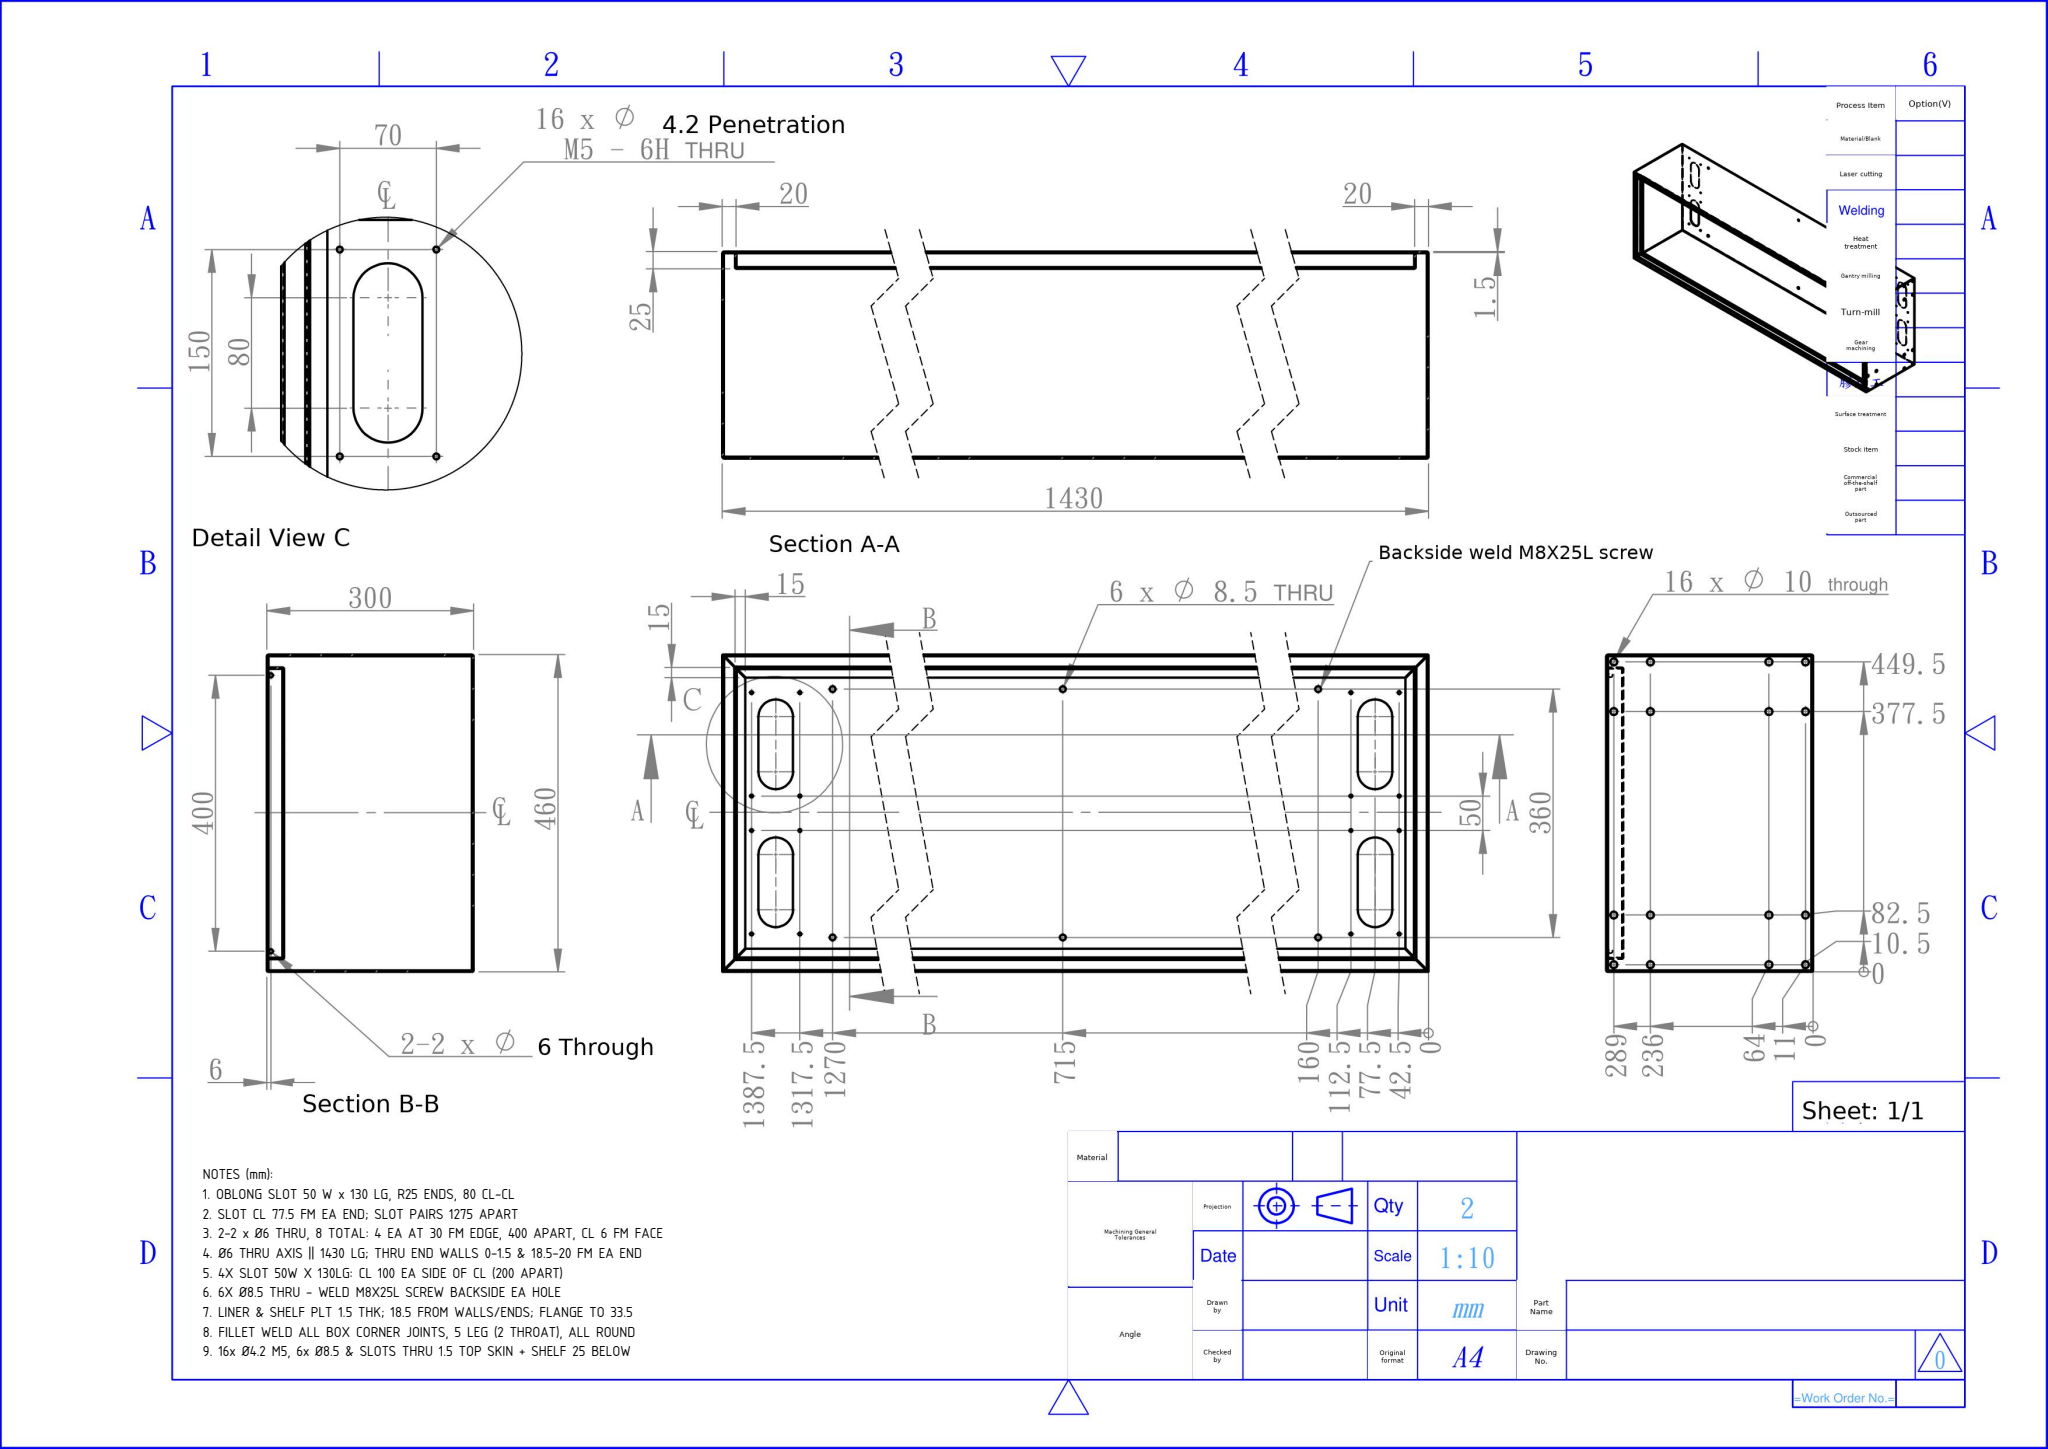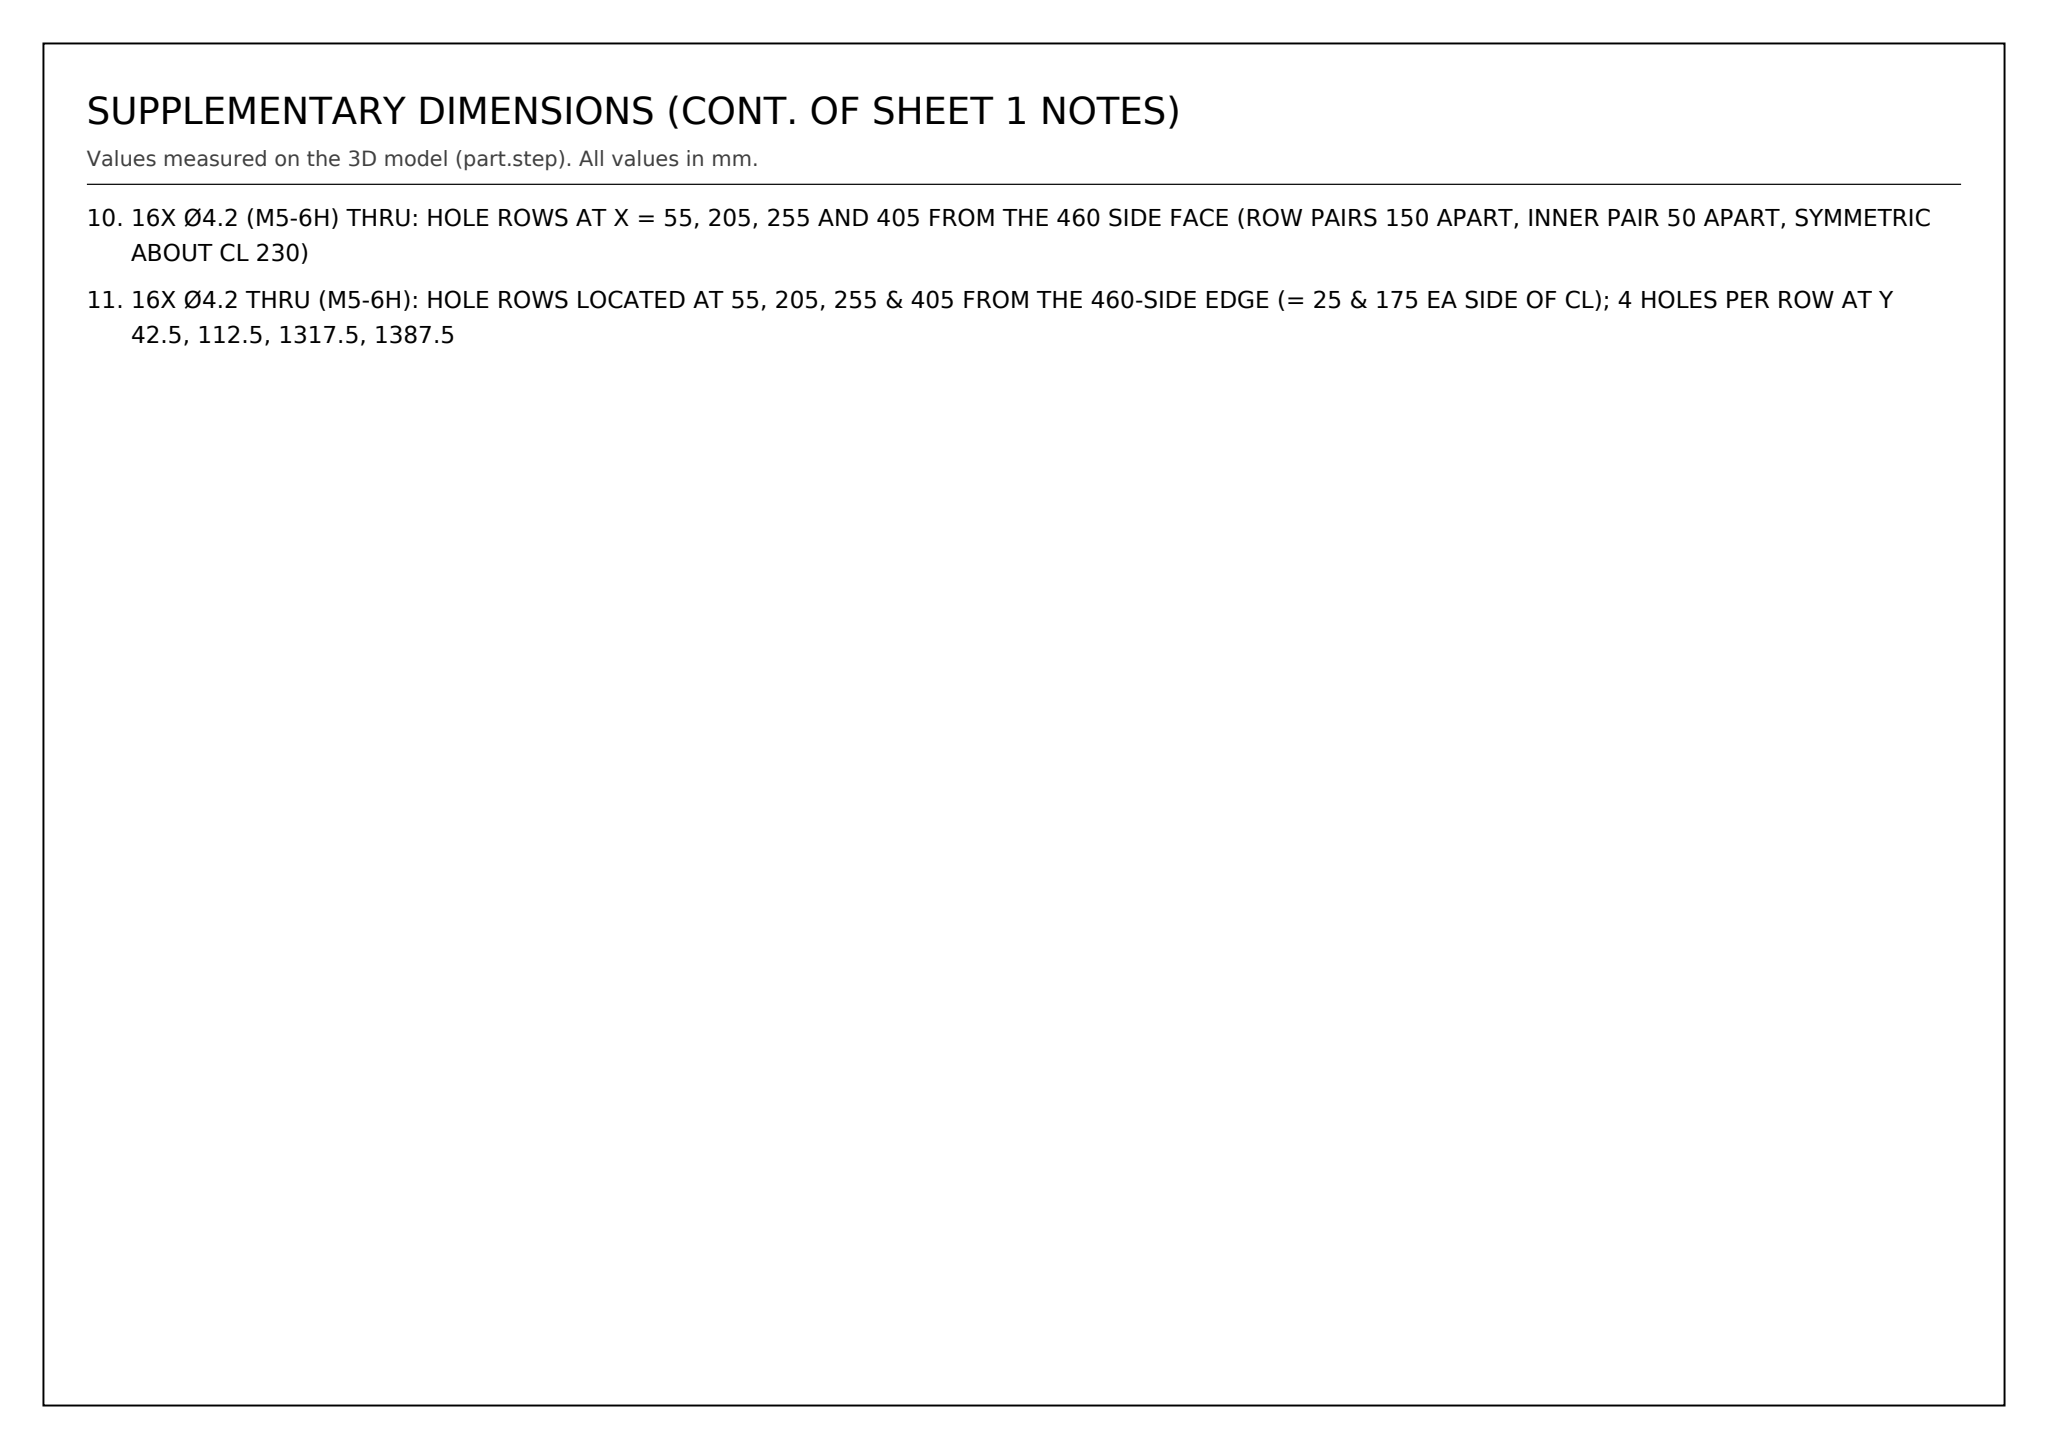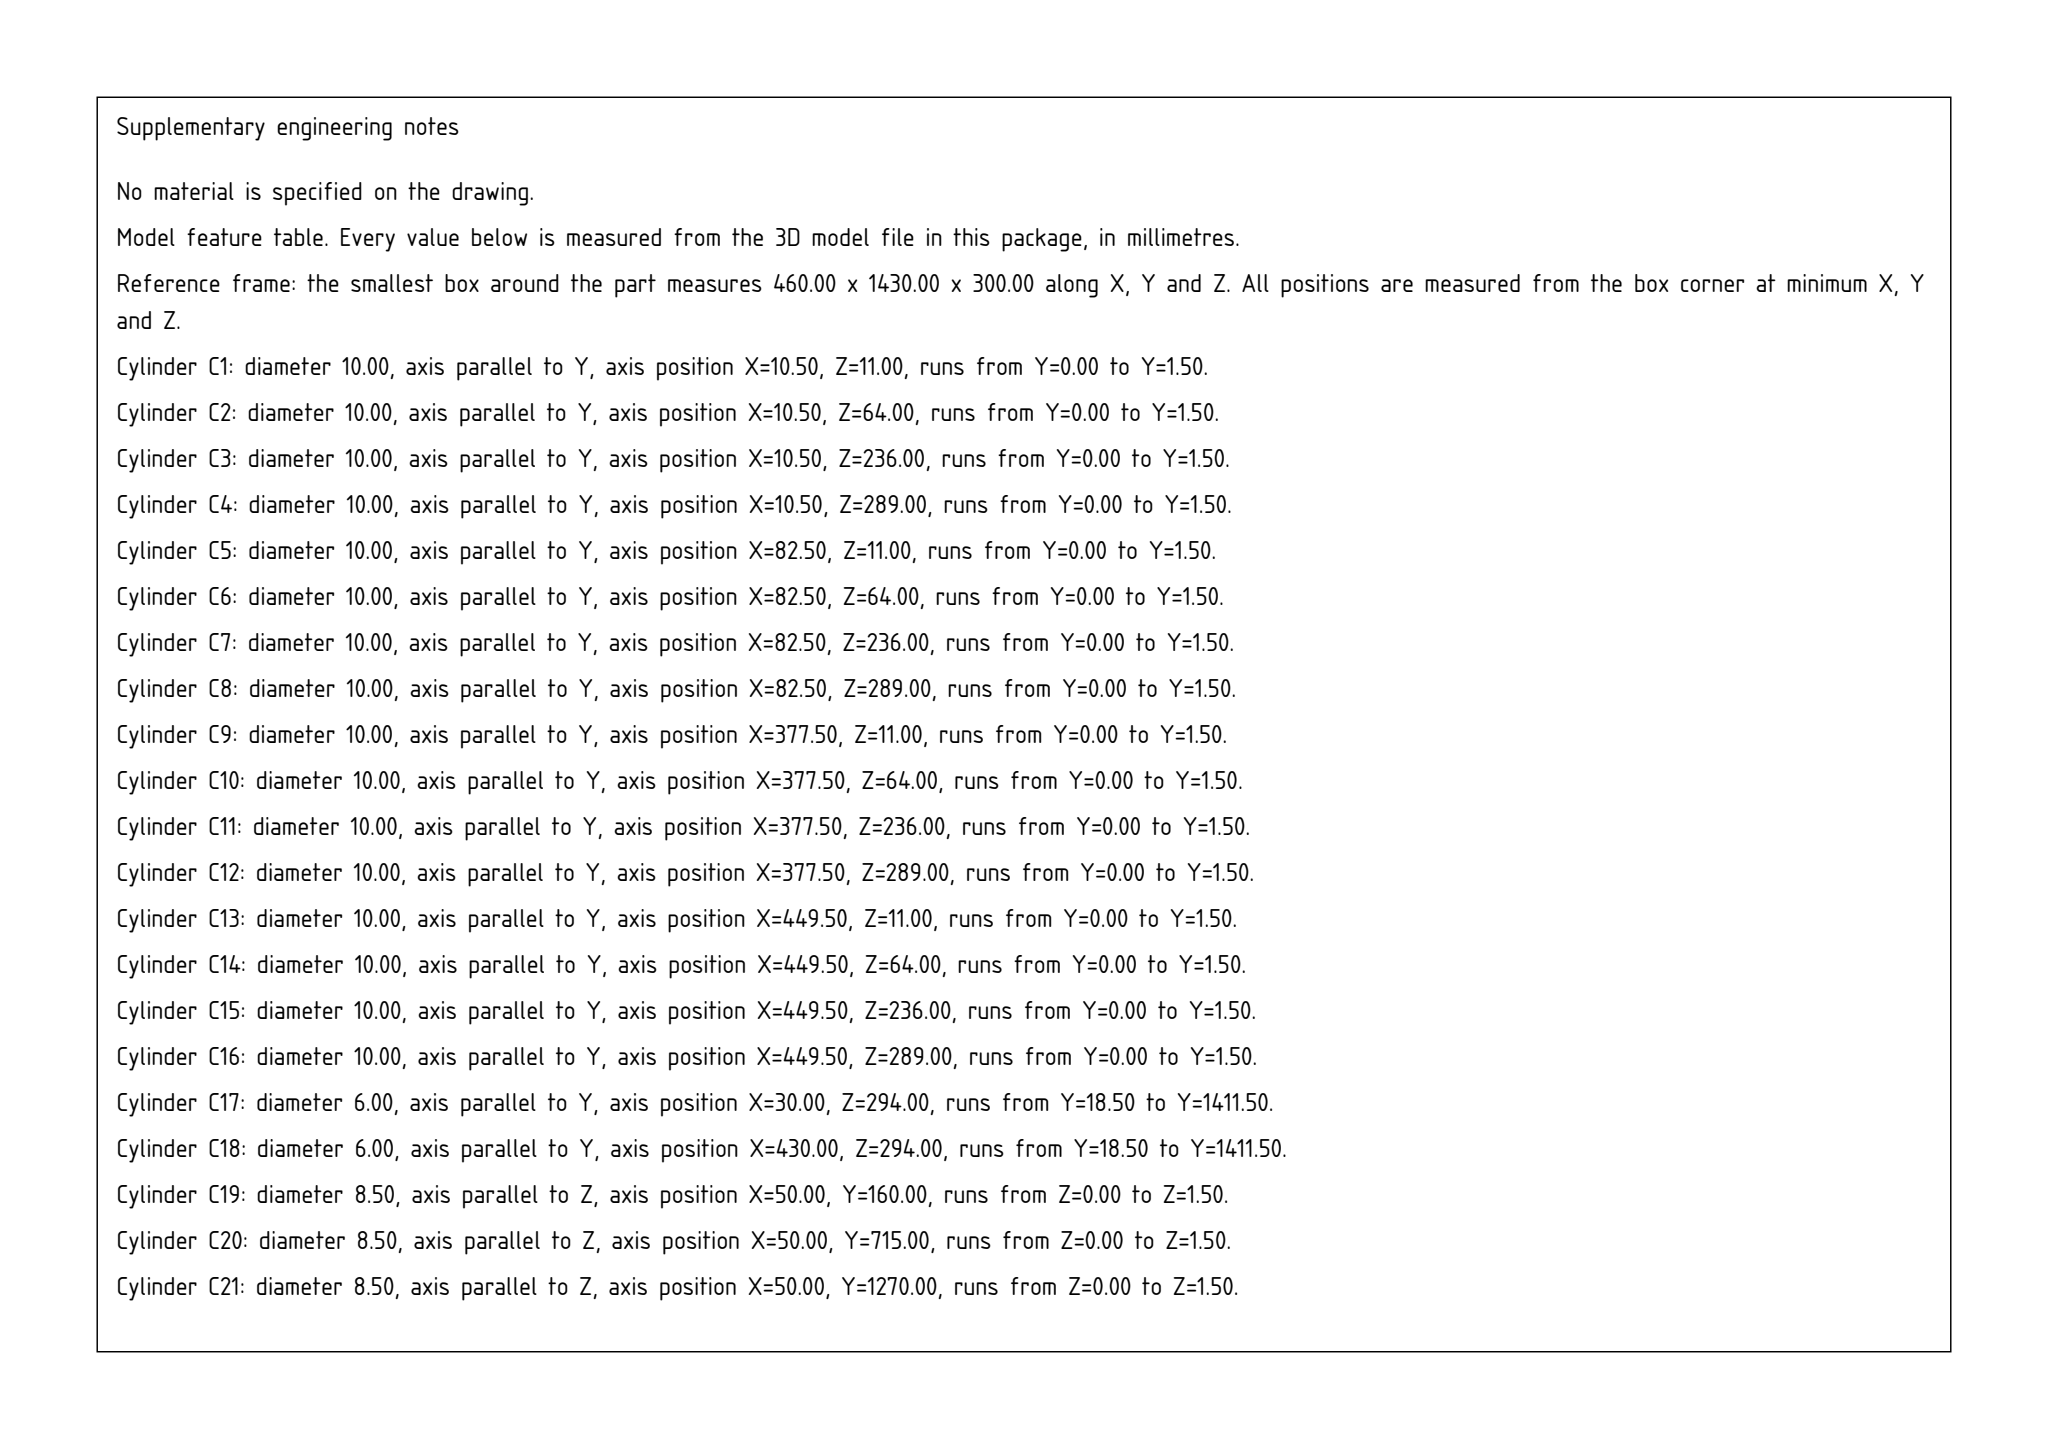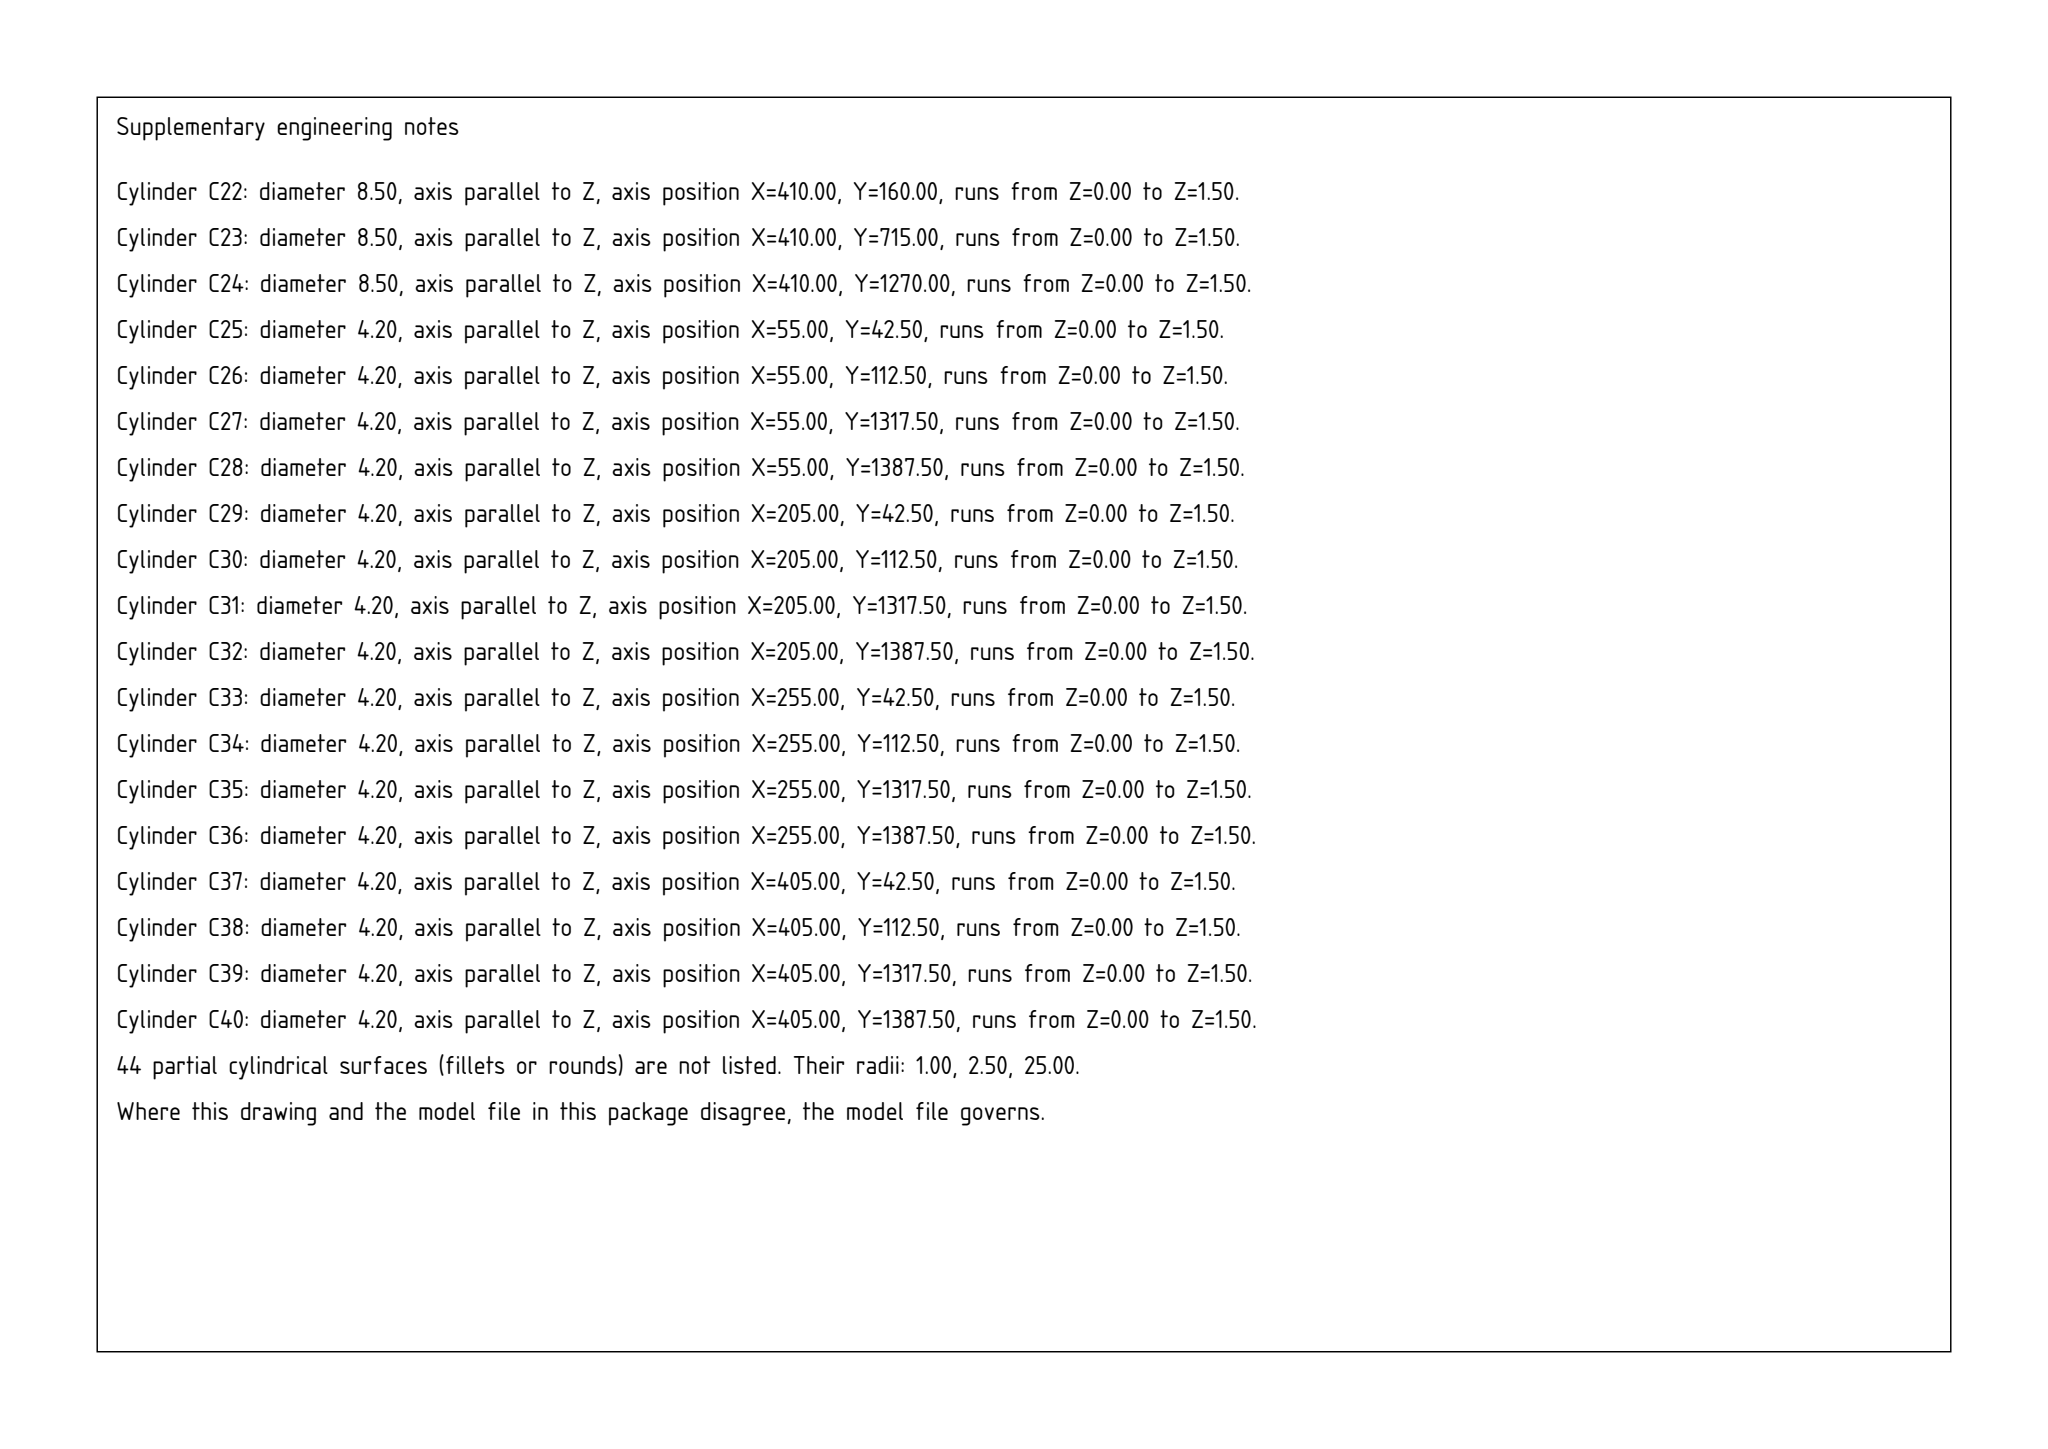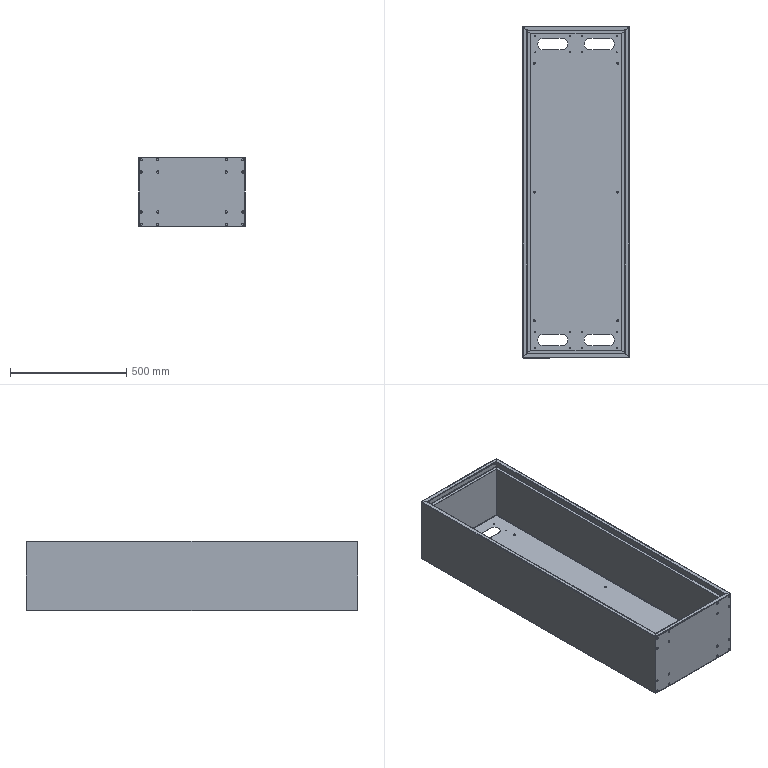Part | SolidWorks | mm | 1 solid | 306 faces | box 460 x 1430 x 300 mm | volume 2922907 mm3 | cylinder 132 | plane 126 | spline 48 | commonest cylinder face diameters 4.2 x32 10 x32 2 x20 5 x16 50 x12 8.5 x12 6 x8
Drawing notes:
OBLONG SLOT 50 W x 130 LG, R25 ENDS, 80 CL-CL | from the solid: Ø50 z-cyls at x=90 & 170 (80 apart); slot side planes y=52.5/102.5 = 50 wide; 80+50=130, R25 ends
SLOT CL 77.5 FM EA END; SLOT PAIRS 1275 APART | from the solid: Ø50 slot end cyls at y=77.5 and y=1352.5; 1430-1352.5=77.5; 1352.5-77.5=1275
2-2 x Ø6 THRU, 8 TOTAL: 4 EA AT 30 FM EDGE, 400 APART, CL 6 FM FACE | from the solid: [6.0,'y',[30,null,294],1.5,4] and [6.0,'y',[430,null,294],1.5,4]; 460-430=30, 430-30=400, 300-294=6
Ø6 THRU AXIS || 1430 LG; THRU END WALLS 0-1.5 & 18.5-20 FM EA END | from the solid: Ø6 cyls axis y, len 1.5; y-planes at 0,1.5,18.5,20 and 1410,1411.5,1428.5,1430
4X SLOT 50W X 130LG: CL 100 EA SIDE OF CL (200 APART) | from the solid: Ø50 end cyls at x=90 & 170 (CL 130) and mirror at x=290 & 370 (CL 330) on 460 width; CL of part = x230, so slots ±100 from ℄, 200 apart; slot W=50, LG=80+50=130
6X Ø8.5 THRU - WELD M8X25L SCREW BACKSIDE EA HOLE | from the solid: Ø8.5 THRU cylinders at (x50,y160),(x50,y715),(x50,y1270),(x410,y160),(x410,y715),(x410,y1270) = 6 holes total
LINER & SHELF PLT 1.5 THK; 18.5 FROM WALLS/ENDS; FLANGE TO 33.5 | from the solid: Planes x/y=18.5,20.0 & 33.5; y=1396.5,1410.0,1411.5; plate faces 1.5 apart (z=275.0/276.5, 298.5/300.0)
FILLET WELD ALL BOX CORNER JOINTS, 5 LEG (2 THROAT), ALL ROUND | from the solid: Ø5 and Ø2 weld-bead cylinders along all 12 corner edges (x,y,z axes, L=1425.59/455.59/295.0)
16x Ø4.2 M5, 6x Ø8.5 & SLOTS THRU 1.5 TOP SKIN + SHELF 25 BELOW | from the solid: Ø4.2, Ø8.5 and 50-wide slot cylinders each L=1.5 with count 2 (top skin z=298.5-300, shelf z=275.0-276.5)
16X Ø4.2 (M5-6H) THRU: HOLE ROWS AT X = 55, 205, 255 AND 405 FROM THE 460 SIDE FACE (ROW PAIRS 150 APART, INNER PAIR 50 APART, SYMMETRIC ABOUT CL 230) | from the solid: cylinders dia 4.2 axis z at x=55.0, 205.0, 255.0, 405.0 (y=42.5/112.5/1317.5/1387.5), length 1.5
16X Ø4.2 THRU (M5-6H): HOLE ROWS LOCATED AT 55, 205, 255 & 405 FROM THE 460-SIDE EDGE (= 25 & 175 EA SIDE OF CL); 4 HOLES PER ROW AT Y 42.5, 112.5, 1317.5, 1387.5 | from the solid: cylinders dia 4.2 axis z at x = 55.0, 205.0, 255.0, 405.0 with y = 42.5, 112.5, 1317.5, 1387.5; bbox_xyz 460 x 1430 x 300